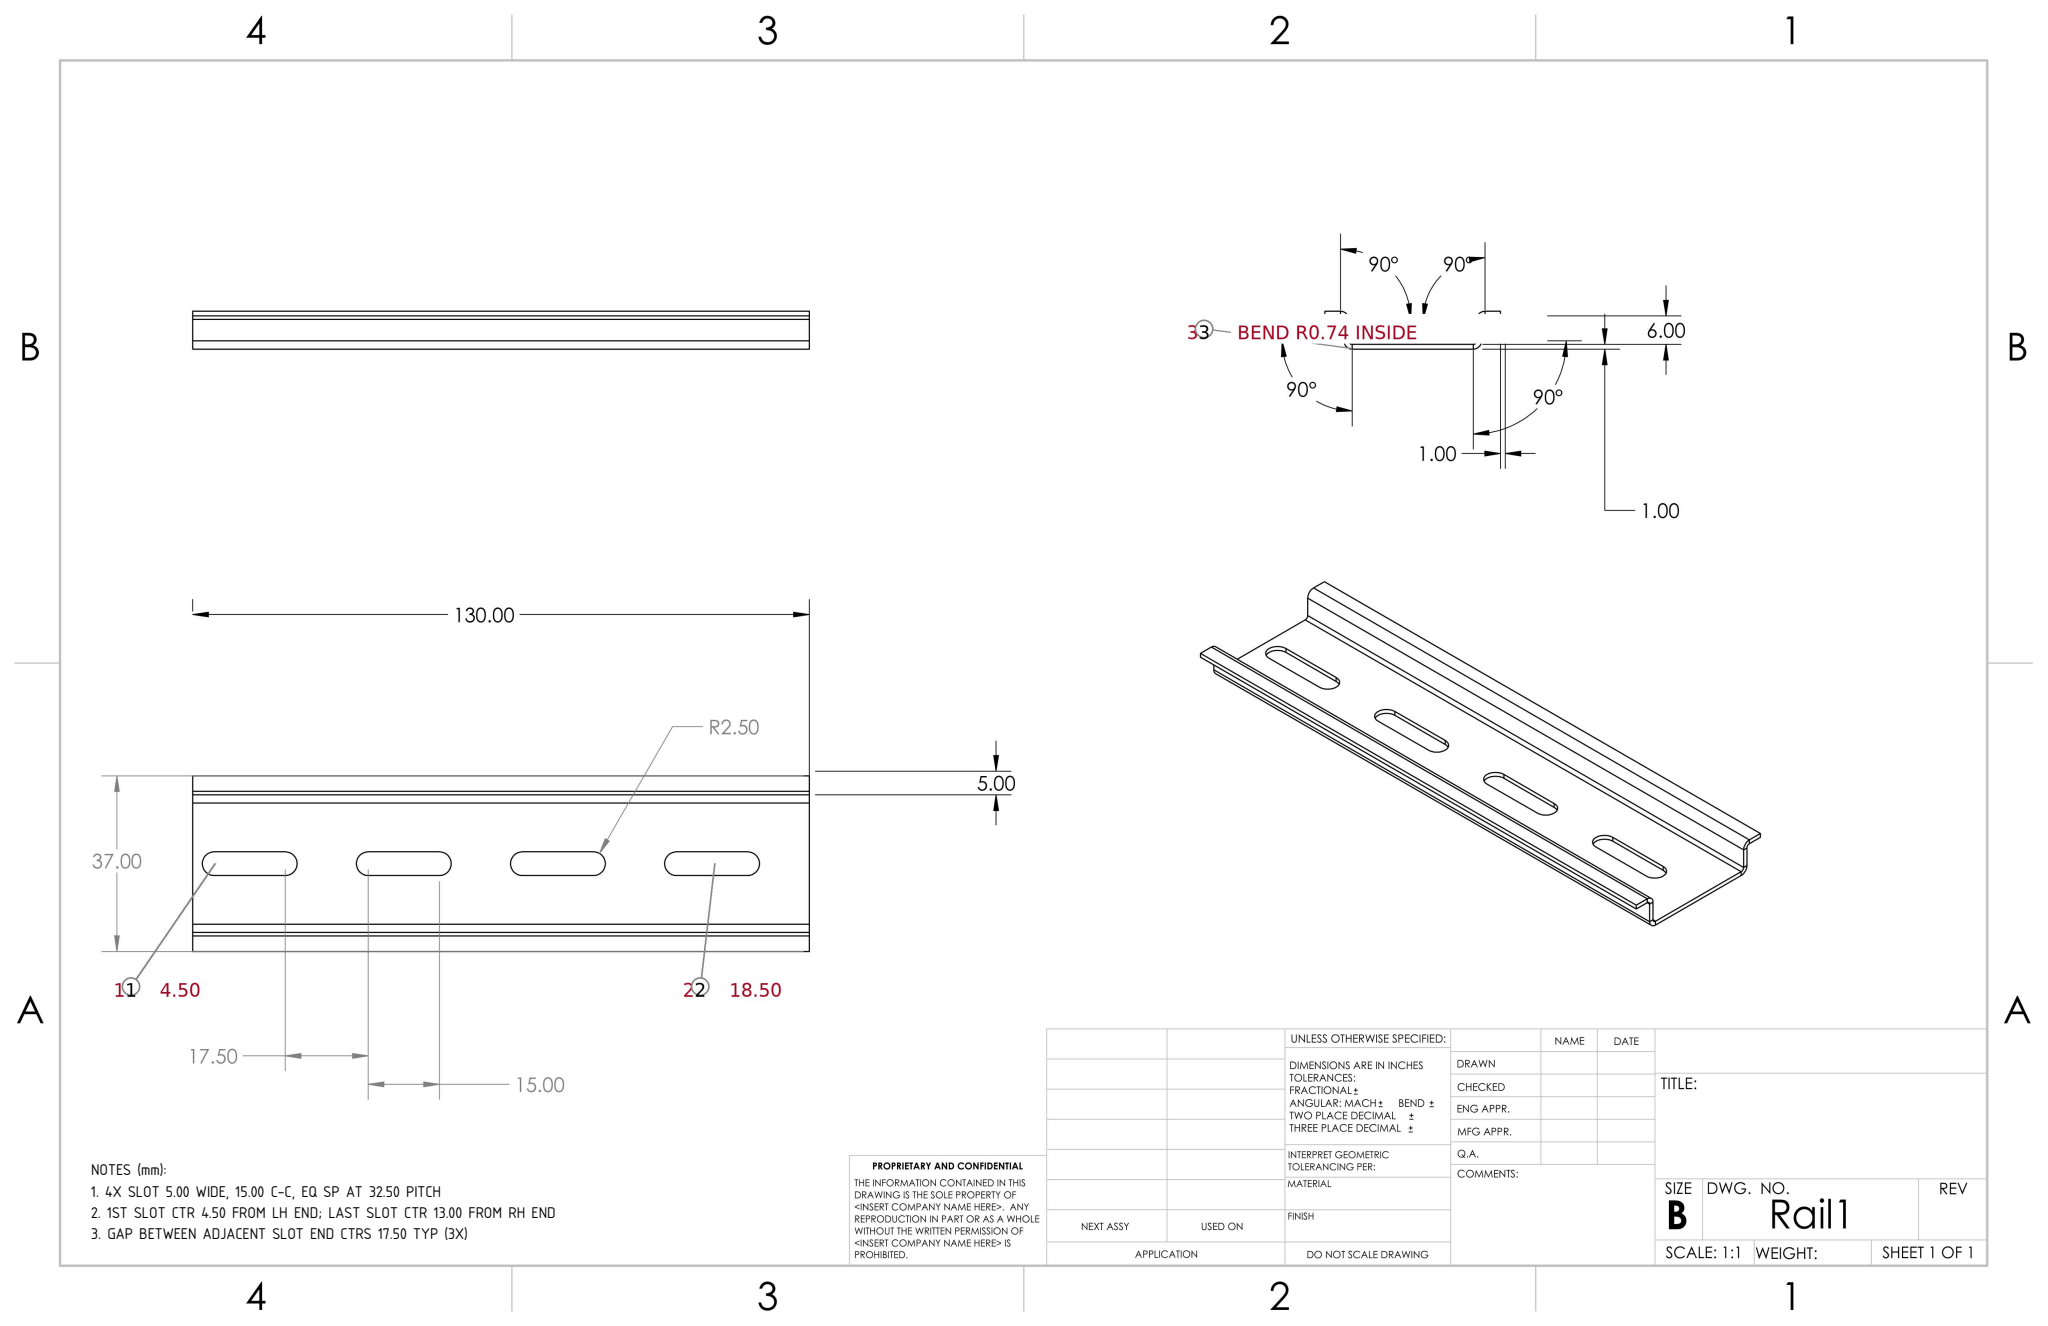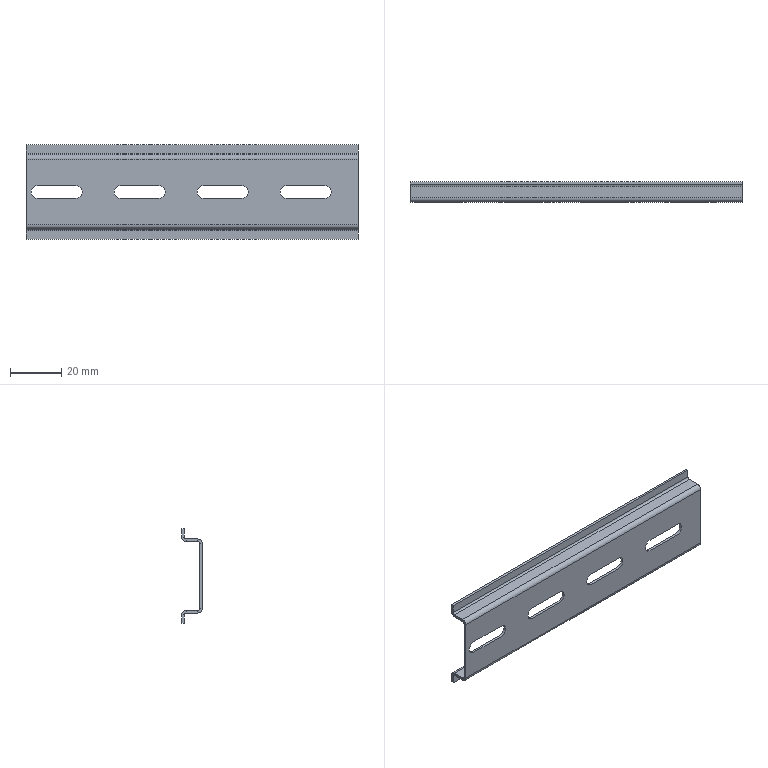Part | SolidWorks | mm | 1 solid | 54 faces | box 130 x 8 x 37 mm | volume 5975 mm3 | plane 38 | cylinder 16 | commonest cylinder face diameters 5 x8 3.473 x4 1.473 x4
Drawing notes:
4X SLOT 5.00 WIDE, 15.00 C-C, EQ SP AT 32.50 PITCH | from the solid: Slot end cyls dia 5.0 at x=4.5/19.5, 37/52, 69.5/84.5, 102/117; 15.0 c-c, pitch 32.5
1ST SLOT CTR 4.50 FROM LH END; LAST SLOT CTR 13.00 FROM RH END | from the solid: First cyl x=4.5; last cyl x=117.0 vs bbox x=130.0 -> 13.0
GAP BETWEEN ADJACENT SLOT END CTRS 17.50 TYP (3X) | from the solid: 37.0-19.5=17.5, 69.5-52.0=17.5, 102.0-84.5=17.5